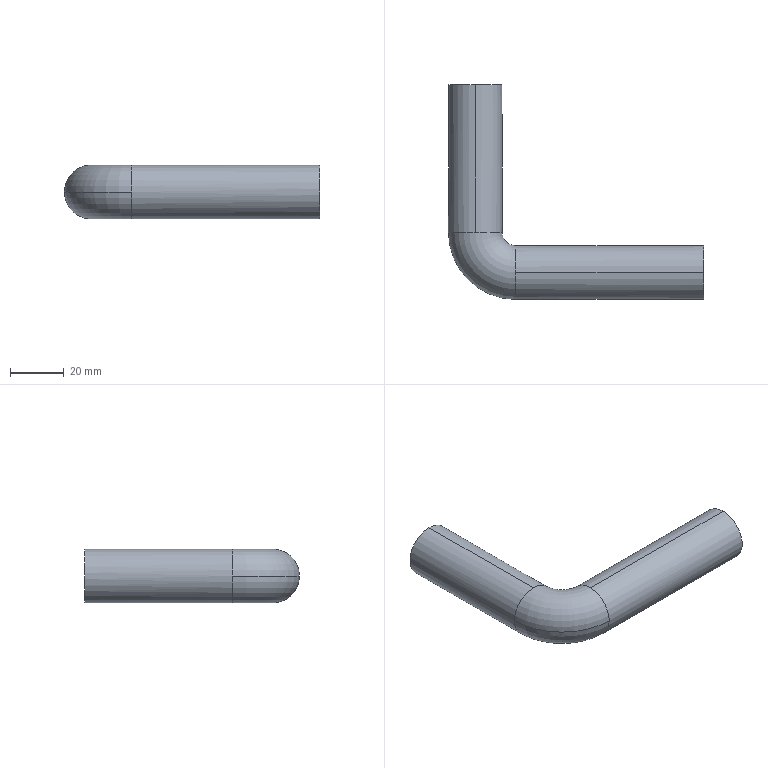Component | SolidWorks | AD12-Handle.SDPRT-5 | 1 solid | 8 faces | box 95 x 80 x 20 mm | volume 46672 mm3 | cylinder 4 | torus 2 | plane 2 | commonest cylinder face diameters 20 x4
build123d program:
from build123d import *

# Parameters (mm, degrees)
SKETCH1_R = 10


with BuildPart() as part:
    # Sweep2: sweep along a path in Sketch2
    with BuildLine(Plane.XY) as sweep2_path:
        Line((0, 0), (-70, 0))
        ThreePointArc((-70, 0), (-80.607, 4.393), (-85, 15))
        Line((-85, 15), (-85, 70))
    # Sketch1 → Sweep2 (sweep)
    with BuildSketch(Plane(origin=(0, 0, 0), x_dir=(0, 0, -1), z_dir=(1, 0, 0))):
        Circle(SKETCH1_R)
    sweep(path=sweep2_path.line)


solid = part.part

# Placed as in the assembly
solid = solid.moved(Location((-179.414, -258.961, 239.12), (0, 0, 0)))
STEP:
#1=COLOUR_RGB('',0.7922,0.8196,0.9333);
#2=FILL_AREA_STYLE_COLOUR('',#1);
#3=FILL_AREA_STYLE('',(#2));
#4=SURFACE_STYLE_FILL_AREA(#3);
#5=SURFACE_SIDE_STYLE('',(#4));
#6=SURFACE_STYLE_USAGE(.BOTH.,#5);
#7=PRESENTATION_STYLE_ASSIGNMENT((#6));
#8=CARTESIAN_POINT('',(-9.819,-10.589,9.414));
#9=VERTEX_POINT('',#8);
#10=CARTESIAN_POINT('',(-9.819,-10.195,9.02));
#11=VERTEX_POINT('',#10);
#12=CARTESIAN_POINT('',(-9.819,-10.195,9.414));
#13=DIRECTION('',(1.,0.,0.));
#14=DIRECTION('',(0.,0.,-1.));
#15=AXIS2_PLACEMENT_3D('',#12,#13,#14);
#16=CIRCLE('',#15,0.3937);
#17=EDGE_CURVE('',#9,#11,#16,.T.);
#18=ORIENTED_EDGE('',*,*,#17,.F.);
#19=CARTESIAN_POINT('',(-10.804,-9.605,9.414));
#20=VERTEX_POINT('',#19);
#21=CARTESIAN_POINT('',(-9.819,-9.605,9.414));
#22=DIRECTION('',(0.,0.,-1.));
#23=DIRECTION('',(-1.,0.,0.));
#24=AXIS2_PLACEMENT_3D('',#21,#22,#23);
#25=CIRCLE('',#24,0.9843);
#26=EDGE_CURVE('',#9,#20,#25,.T.);
#27=ORIENTED_EDGE('',*,*,#26,.T.);
#28=CARTESIAN_POINT('',(-10.41,-9.605,9.02));
#29=VERTEX_POINT('',#28);
#30=CARTESIAN_POINT('',(-10.41,-9.605,9.414));
#31=DIRECTION('',(0.,-1.,0.));
#32=DIRECTION('',(0.,0.,-1.));
#33=AXIS2_PLACEMENT_3D('',#30,#31,#32);
#34=CIRCLE('',#33,0.3937);
#35=EDGE_CURVE('',#20,#29,#34,.T.);
#36=ORIENTED_EDGE('',*,*,#35,.T.);
#37=CARTESIAN_POINT('',(-10.016,-9.605,9.414));
#38=VERTEX_POINT('',#37);
#39=CARTESIAN_POINT('',(-10.41,-9.605,9.414));
#40=DIRECTION('',(0.,-1.,0.));
#41=DIRECTION('',(0.,0.,-1.));
#42=AXIS2_PLACEMENT_3D('',#39,#40,#41);
#43=CIRCLE('',#42,0.3937);
#44=EDGE_CURVE('',#29,#38,#43,.T.);
#45=ORIENTED_EDGE('',*,*,#44,.T.);
#46=CARTESIAN_POINT('',(-9.819,-9.802,9.414));
#47=VERTEX_POINT('',#46);
#48=CARTESIAN_POINT('',(-9.819,-9.605,9.414));
#49=DIRECTION('',(0.,0.,-1.));
#50=DIRECTION('',(-1.,0.,0.));
#51=AXIS2_PLACEMENT_3D('',#48,#49,#50);
#52=CIRCLE('',#51,0.1969);
#53=EDGE_CURVE('',#47,#38,#52,.T.);
#54=ORIENTED_EDGE('',*,*,#53,.F.);
#55=CARTESIAN_POINT('',(-9.819,-10.195,9.414));
#56=DIRECTION('',(1.,0.,0.));
#57=DIRECTION('',(0.,0.,-1.));
#58=AXIS2_PLACEMENT_3D('',#55,#56,#57);
#59=CIRCLE('',#58,0.3937);
#60=EDGE_CURVE('',#11,#47,#59,.T.);
#61=ORIENTED_EDGE('',*,*,#60,.F.);
#62=EDGE_LOOP('',(#18,#27,#36,#45,#54,#61));
#63=FACE_OUTER_BOUND('',#62,.T.);
#64=CARTESIAN_POINT('',(-9.819,-9.605,9.414));
#65=DIRECTION('',(0.,0.,-1.));
#66=DIRECTION('',(-1.,0.,0.));
#67=AXIS2_PLACEMENT_3D('',#64,#65,#66);
#68=TOROIDAL_SURFACE('',#67,0.5906,0.3937);
#69=ADVANCED_FACE('',(#63),#68,.T.);
#70=ORIENTED_EDGE('',*,*,#60,.T.);
#71=CARTESIAN_POINT('',(-9.819,-10.195,9.808));
#72=VERTEX_POINT('',#71);
#73=CARTESIAN_POINT('',(-9.819,-10.195,9.414));
#74=DIRECTION('',(1.,0.,0.));
#75=DIRECTION('',(0.,0.,-1.));
#76=AXIS2_PLACEMENT_3D('',#73,#74,#75);
#77=CIRCLE('',#76,0.3937);
#78=EDGE_CURVE('',#47,#72,#77,.T.);
#79=ORIENTED_EDGE('',*,*,#78,.T.);
#80=CARTESIAN_POINT('',(-7.064,-10.195,9.808));
#81=VERTEX_POINT('',#80);
#82=CARTESIAN_POINT('',(-9.819,-10.195,9.808));
#83=DIRECTION('',(1.,0.,0.));
#84=VECTOR('',#83,39.37);
#85=LINE('',#82,#84);
#86=EDGE_CURVE('',#72,#81,#85,.T.);
#87=ORIENTED_EDGE('',*,*,#86,.T.);
#88=CARTESIAN_POINT('',(-7.064,-10.195,9.02));
#89=VERTEX_POINT('',#88);
#90=CARTESIAN_POINT('',(-7.064,-10.195,9.414));
#91=DIRECTION('',(1.,0.,0.));
#92=DIRECTION('',(0.,0.,-1.));
#93=AXIS2_PLACEMENT_3D('',#90,#91,#92);
#94=CIRCLE('',#93,0.3937);
#95=EDGE_CURVE('',#89,#81,#94,.T.);
#96=ORIENTED_EDGE('',*,*,#95,.F.);
#97=CARTESIAN_POINT('',(-9.819,-10.195,9.02));
#98=DIRECTION('',(1.,0.,0.));
#99=VECTOR('',#98,39.37);
#100=LINE('',#97,#99);
#101=EDGE_CURVE('',#11,#89,#100,.T.);
#102=ORIENTED_EDGE('',*,*,#101,.F.);
#103=EDGE_LOOP('',(#70,#79,#87,#96,#102));
#104=FACE_OUTER_BOUND('',#103,.T.);
#105=CARTESIAN_POINT('',(-9.819,-10.195,9.414));
#106=DIRECTION('',(1.,0.,0.));
#107=DIRECTION('',(0.,0.,-1.));
#108=AXIS2_PLACEMENT_3D('',#105,#106,#107);
#109=CYLINDRICAL_SURFACE('',#108,0.3937);
#110=ADVANCED_FACE('',(#104),#109,.T.);
#111=ORIENTED_EDGE('',*,*,#44,.F.);
#112=CARTESIAN_POINT('',(-10.41,-7.439,9.02));
#113=VERTEX_POINT('',#112);
#114=CARTESIAN_POINT('',(-10.41,-9.605,9.02));
#115=DIRECTION('',(0.,1.,0.));
#116=VECTOR('',#115,39.37);
#117=LINE('',#114,#116);
#118=EDGE_CURVE('',#29,#113,#117,.T.);
#119=ORIENTED_EDGE('',*,*,#118,.T.);
#120=CARTESIAN_POINT('',(-10.41,-7.439,9.808));
#121=VERTEX_POINT('',#120);
#122=CARTESIAN_POINT('',(-10.41,-7.439,9.414));
#123=DIRECTION('',(0.,-1.,0.));
#124=DIRECTION('',(0.,0.,-1.));
#125=AXIS2_PLACEMENT_3D('',#122,#123,#124);
#126=CIRCLE('',#125,0.3937);
#127=EDGE_CURVE('',#113,#121,#126,.T.);
#128=ORIENTED_EDGE('',*,*,#127,.T.);
#129=CARTESIAN_POINT('',(-10.41,-9.605,9.808));
#130=VERTEX_POINT('',#129);
#131=CARTESIAN_POINT('',(-10.41,-9.605,9.808));
#132=DIRECTION('',(0.,1.,0.));
#133=VECTOR('',#132,39.37);
#134=LINE('',#131,#133);
#135=EDGE_CURVE('',#130,#121,#134,.T.);
#136=ORIENTED_EDGE('',*,*,#135,.F.);
#137=CARTESIAN_POINT('',(-10.41,-9.605,9.414));
#138=DIRECTION('',(0.,-1.,0.));
#139=DIRECTION('',(0.,0.,-1.));
#140=AXIS2_PLACEMENT_3D('',#137,#138,#139);
#141=CIRCLE('',#140,0.3937);
#142=EDGE_CURVE('',#38,#130,#141,.T.);
#143=ORIENTED_EDGE('',*,*,#142,.F.);
#144=EDGE_LOOP('',(#111,#119,#128,#136,#143));
#145=FACE_OUTER_BOUND('',#144,.T.);
#146=CARTESIAN_POINT('',(-10.41,-9.605,9.414));
#147=DIRECTION('',(0.,1.,0.));
#148=DIRECTION('',(0.,0.,1.));
#149=AXIS2_PLACEMENT_3D('',#146,#147,#148);
#150=CYLINDRICAL_SURFACE('',#149,0.3937);
#151=ADVANCED_FACE('',(#145),#150,.T.);
#152=ORIENTED_EDGE('',*,*,#118,.F.);
#153=ORIENTED_EDGE('',*,*,#35,.F.);
#154=CARTESIAN_POINT('',(-10.41,-9.605,9.414));
#155=DIRECTION('',(0.,-1.,0.));
#156=DIRECTION('',(0.,0.,-1.));
#157=AXIS2_PLACEMENT_3D('',#154,#155,#156);
#158=CIRCLE('',#157,0.3937);
#159=EDGE_CURVE('',#130,#20,#158,.T.);
#160=ORIENTED_EDGE('',*,*,#159,.F.);
#161=ORIENTED_EDGE('',*,*,#135,.T.);
#162=CARTESIAN_POINT('',(-10.41,-7.439,9.414));
#163=DIRECTION('',(0.,-1.,0.));
#164=DIRECTION('',(0.,0.,-1.));
#165=AXIS2_PLACEMENT_3D('',#162,#163,#164);
#166=CIRCLE('',#165,0.3937);
#167=EDGE_CURVE('',#121,#113,#166,.T.);
#168=ORIENTED_EDGE('',*,*,#167,.T.);
#169=EDGE_LOOP('',(#152,#153,#160,#161,#168));
#170=FACE_OUTER_BOUND('',#169,.T.);
#171=CARTESIAN_POINT('',(-10.41,-9.605,9.414));
#172=DIRECTION('',(0.,1.,0.));
#173=DIRECTION('',(0.,0.,1.));
#174=AXIS2_PLACEMENT_3D('',#171,#172,#173);
#175=CYLINDRICAL_SURFACE('',#174,0.3937);
#176=ADVANCED_FACE('',(#170),#175,.T.);
#177=ORIENTED_EDGE('',*,*,#26,.F.);
#178=CARTESIAN_POINT('',(-9.819,-10.195,9.414));
#179=DIRECTION('',(1.,0.,0.));
#180=DIRECTION('',(0.,0.,-1.));
#181=AXIS2_PLACEMENT_3D('',#178,#179,#180);
#182=CIRCLE('',#181,0.3937);
#183=EDGE_CURVE('',#72,#9,#182,.T.);
#184=ORIENTED_EDGE('',*,*,#183,.F.);
#185=ORIENTED_EDGE('',*,*,#78,.F.);
#186=ORIENTED_EDGE('',*,*,#53,.T.);
#187=ORIENTED_EDGE('',*,*,#142,.T.);
#188=ORIENTED_EDGE('',*,*,#159,.T.);
#189=EDGE_LOOP('',(#177,#184,#185,#186,#187,#188));
#190=FACE_OUTER_BOUND('',#189,.T.);
#191=CARTESIAN_POINT('',(-9.819,-9.605,9.414));
#192=DIRECTION('',(0.,0.,-1.));
#193=DIRECTION('',(-1.,0.,0.));
#194=AXIS2_PLACEMENT_3D('',#191,#192,#193);
#195=TOROIDAL_SURFACE('',#194,0.5906,0.3937);
#196=ADVANCED_FACE('',(#190),#195,.T.);
#197=ORIENTED_EDGE('',*,*,#86,.F.);
#198=ORIENTED_EDGE('',*,*,#183,.T.);
#199=ORIENTED_EDGE('',*,*,#17,.T.);
#200=ORIENTED_EDGE('',*,*,#101,.T.);
#201=CARTESIAN_POINT('',(-7.064,-10.195,9.414));
#202=DIRECTION('',(1.,0.,0.));
#203=DIRECTION('',(0.,0.,-1.));
#204=AXIS2_PLACEMENT_3D('',#201,#202,#203);
#205=CIRCLE('',#204,0.3937);
#206=EDGE_CURVE('',#81,#89,#205,.T.);
#207=ORIENTED_EDGE('',*,*,#206,.F.);
#208=EDGE_LOOP('',(#197,#198,#199,#200,#207));
#209=FACE_OUTER_BOUND('',#208,.T.);
#210=CARTESIAN_POINT('',(-9.819,-10.195,9.414));
#211=DIRECTION('',(1.,0.,0.));
#212=DIRECTION('',(0.,0.,-1.));
#213=AXIS2_PLACEMENT_3D('',#210,#211,#212);
#214=CYLINDRICAL_SURFACE('',#213,0.3937);
#215=ADVANCED_FACE('',(#209),#214,.T.);
#216=ORIENTED_EDGE('',*,*,#167,.F.);
#217=ORIENTED_EDGE('',*,*,#127,.F.);
#218=EDGE_LOOP('',(#216,#217));
#219=FACE_OUTER_BOUND('',#218,.T.);
#220=CARTESIAN_POINT('',(-10.41,-7.439,9.414));
#221=DIRECTION('',(0.,-1.,0.));
#222=DIRECTION('',(0.,0.,-1.));
#223=AXIS2_PLACEMENT_3D('',#220,#221,#222);
#224=PLANE('',#223);
#225=ADVANCED_FACE('',(#219),#224,.F.);
#226=ORIENTED_EDGE('',*,*,#95,.T.);
#227=ORIENTED_EDGE('',*,*,#206,.T.);
#228=EDGE_LOOP('',(#226,#227));
#229=FACE_OUTER_BOUND('',#228,.T.);
#230=CARTESIAN_POINT('',(-7.064,-10.195,9.414));
#231=DIRECTION('',(1.,0.,0.));
#232=DIRECTION('',(0.,0.,-1.));
#233=AXIS2_PLACEMENT_3D('',#230,#231,#232);
#234=PLANE('',#233);
#235=ADVANCED_FACE('',(#229),#234,.T.);
#236=CLOSED_SHELL('',(#69,#110,#151,#176,#196,#215,#225,#235));
#237=MANIFOLD_SOLID_BREP('',#236);
#238=STYLED_ITEM('',(#7),#237);
#239=(LENGTH_UNIT()NAMED_UNIT(*)SI_UNIT($,.METRE.));
#240=LENGTH_MEASURE_WITH_UNIT(LENGTH_MEASURE(0.0254),#239);
#241=DIMENSIONAL_EXPONENTS(1.,0.,0.,0.,0.,0.,0.);
#242=(CONVERSION_BASED_UNIT('',#240)LENGTH_UNIT()NAMED_UNIT(#241));
#243=UNCERTAINTY_MEASURE_WITH_UNIT(LENGTH_MEASURE(0.00001),#242,'','');
#244=(NAMED_UNIT(*)PLANE_ANGLE_UNIT()SI_UNIT($,.RADIAN.));
#245=(NAMED_UNIT(*)SI_UNIT($,.STERADIAN.)SOLID_ANGLE_UNIT());
#246=(GEOMETRIC_REPRESENTATION_CONTEXT(3)GLOBAL_UNCERTAINTY_ASSIGNED_CONTEXT((#243))GLOBAL_UNIT_ASSIGNED_CONTEXT((#242,#244,#245))REPRESENTATION_CONTEXT('',''));
#247=MECHANICAL_DESIGN_GEOMETRIC_PRESENTATION_REPRESENTATION('',(#238),#246);
#248=PRESENTATION_LAYER_ASSIGNMENT('','',(#238));
#249=CARTESIAN_POINT('',(0.,0.,0.));
#250=DIRECTION('',(0.,0.,1.));
#251=DIRECTION('',(1.,0.,0.));
#252=AXIS2_PLACEMENT_3D('',#249,#250,#251);
#253=(LENGTH_UNIT()NAMED_UNIT(*)SI_UNIT($,.METRE.));
#254=LENGTH_MEASURE_WITH_UNIT(LENGTH_MEASURE(0.0254),#253);
#255=DIMENSIONAL_EXPONENTS(1.,0.,0.,0.,0.,0.,0.);
#256=(CONVERSION_BASED_UNIT('',#254)LENGTH_UNIT()NAMED_UNIT(#255));
#257=UNCERTAINTY_MEASURE_WITH_UNIT(LENGTH_MEASURE(0.00001),#256,'','');
#258=(NAMED_UNIT(*)PLANE_ANGLE_UNIT()SI_UNIT($,.RADIAN.));
#259=(NAMED_UNIT(*)SI_UNIT($,.STERADIAN.)SOLID_ANGLE_UNIT());
#260=(GEOMETRIC_REPRESENTATION_CONTEXT(3)GLOBAL_UNCERTAINTY_ASSIGNED_CONTEXT((#257))GLOBAL_UNIT_ASSIGNED_CONTEXT((#256,#258,#259))REPRESENTATION_CONTEXT('',''));
#261=ADVANCED_BREP_SHAPE_REPRESENTATION('',(#237,#252),#260);